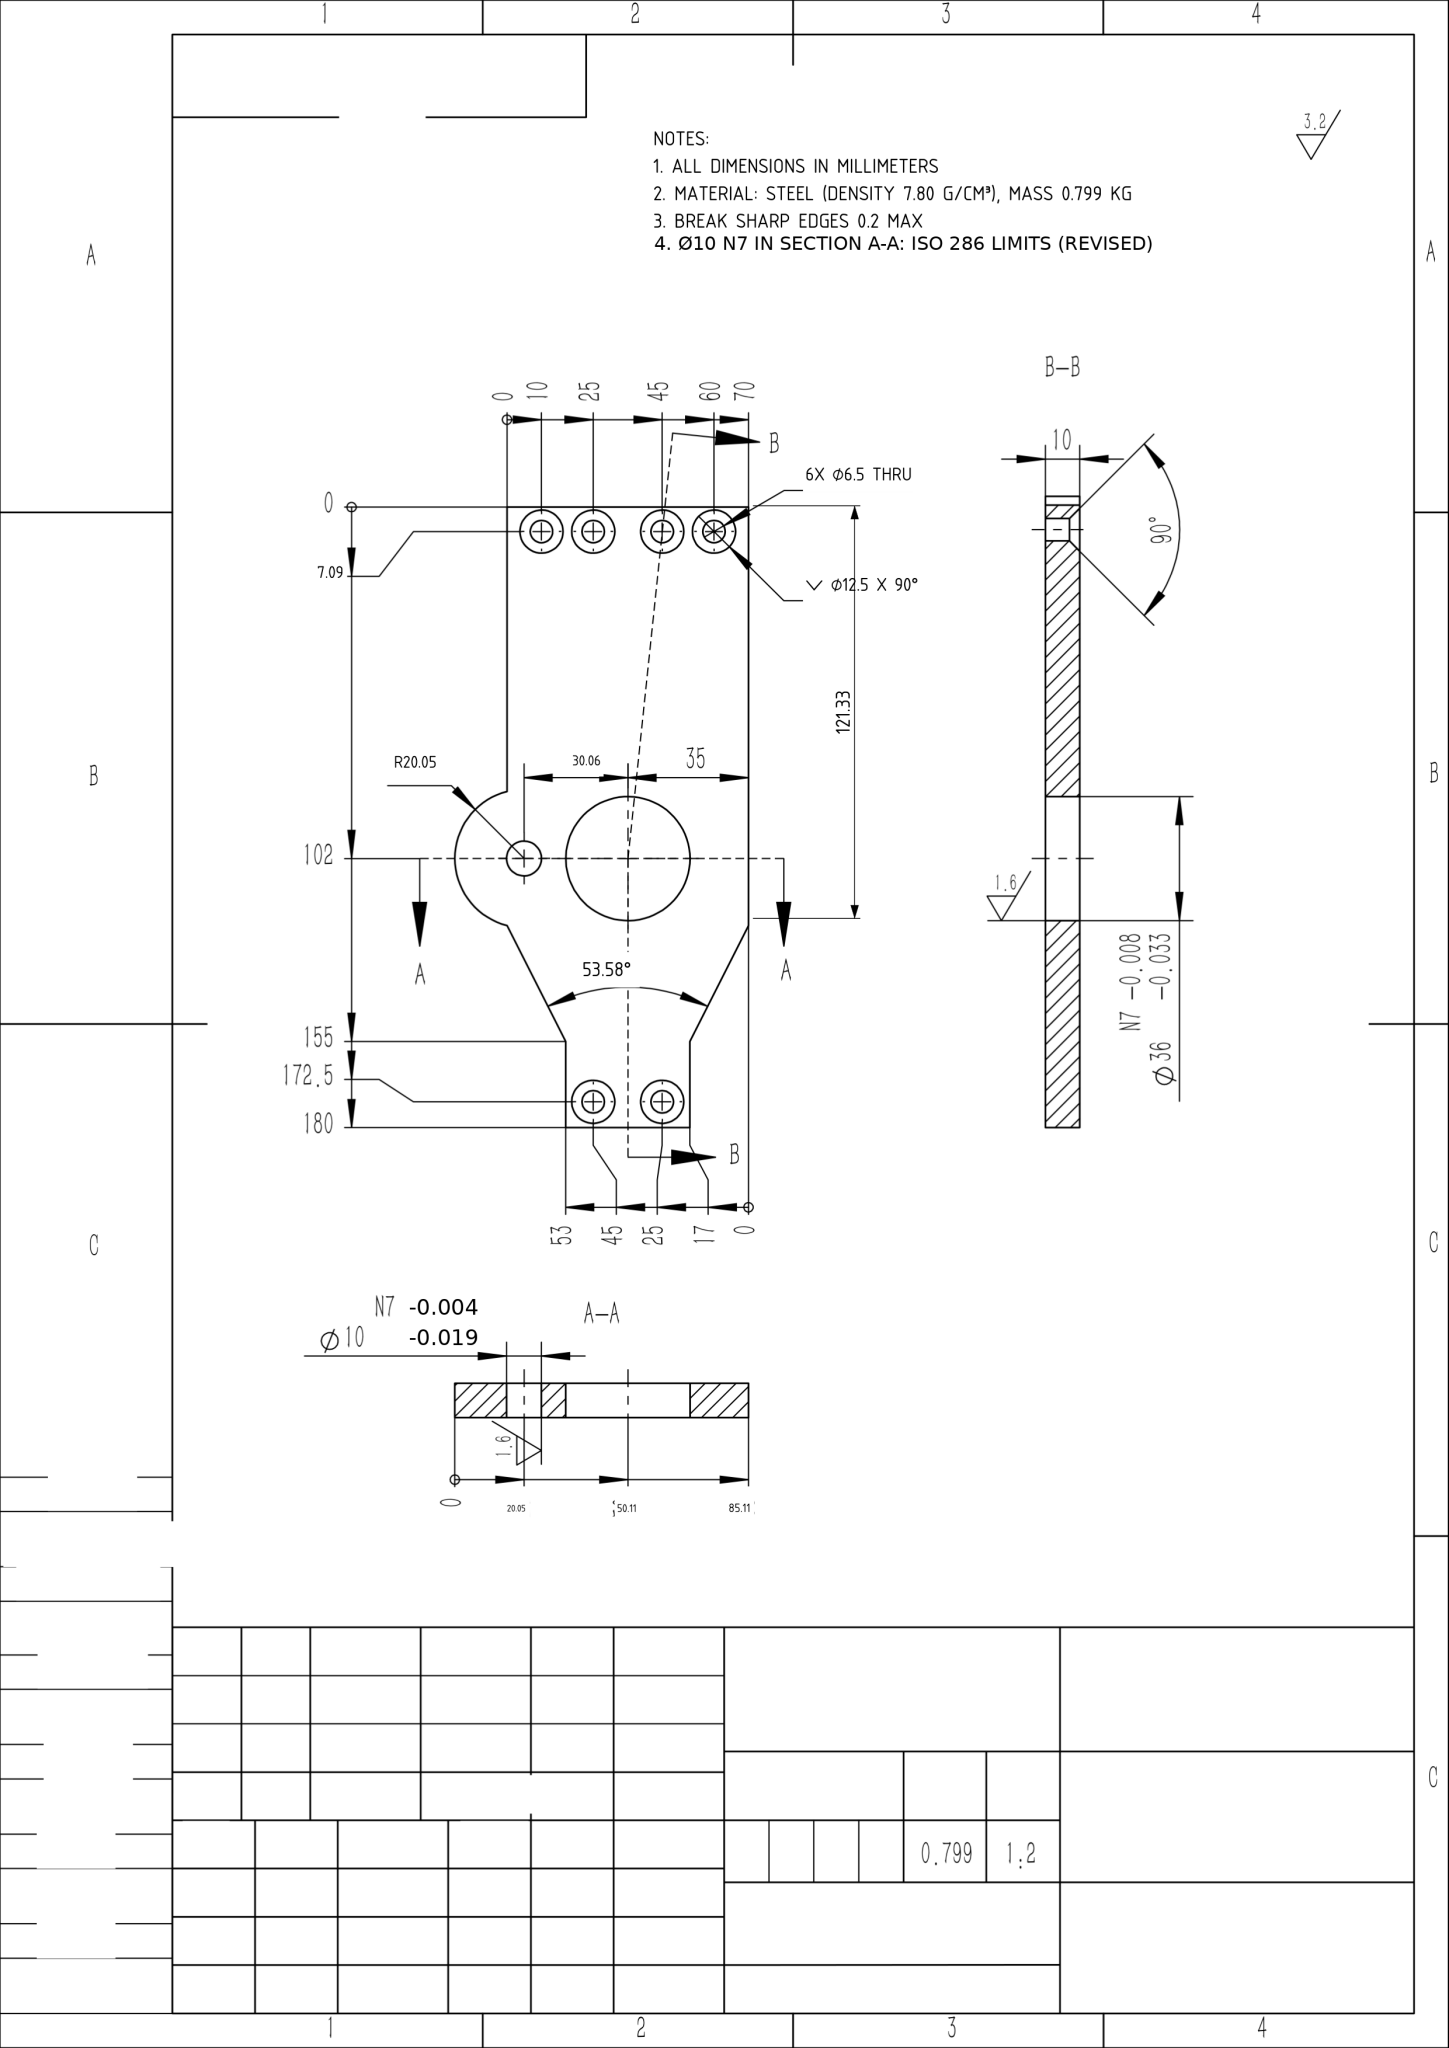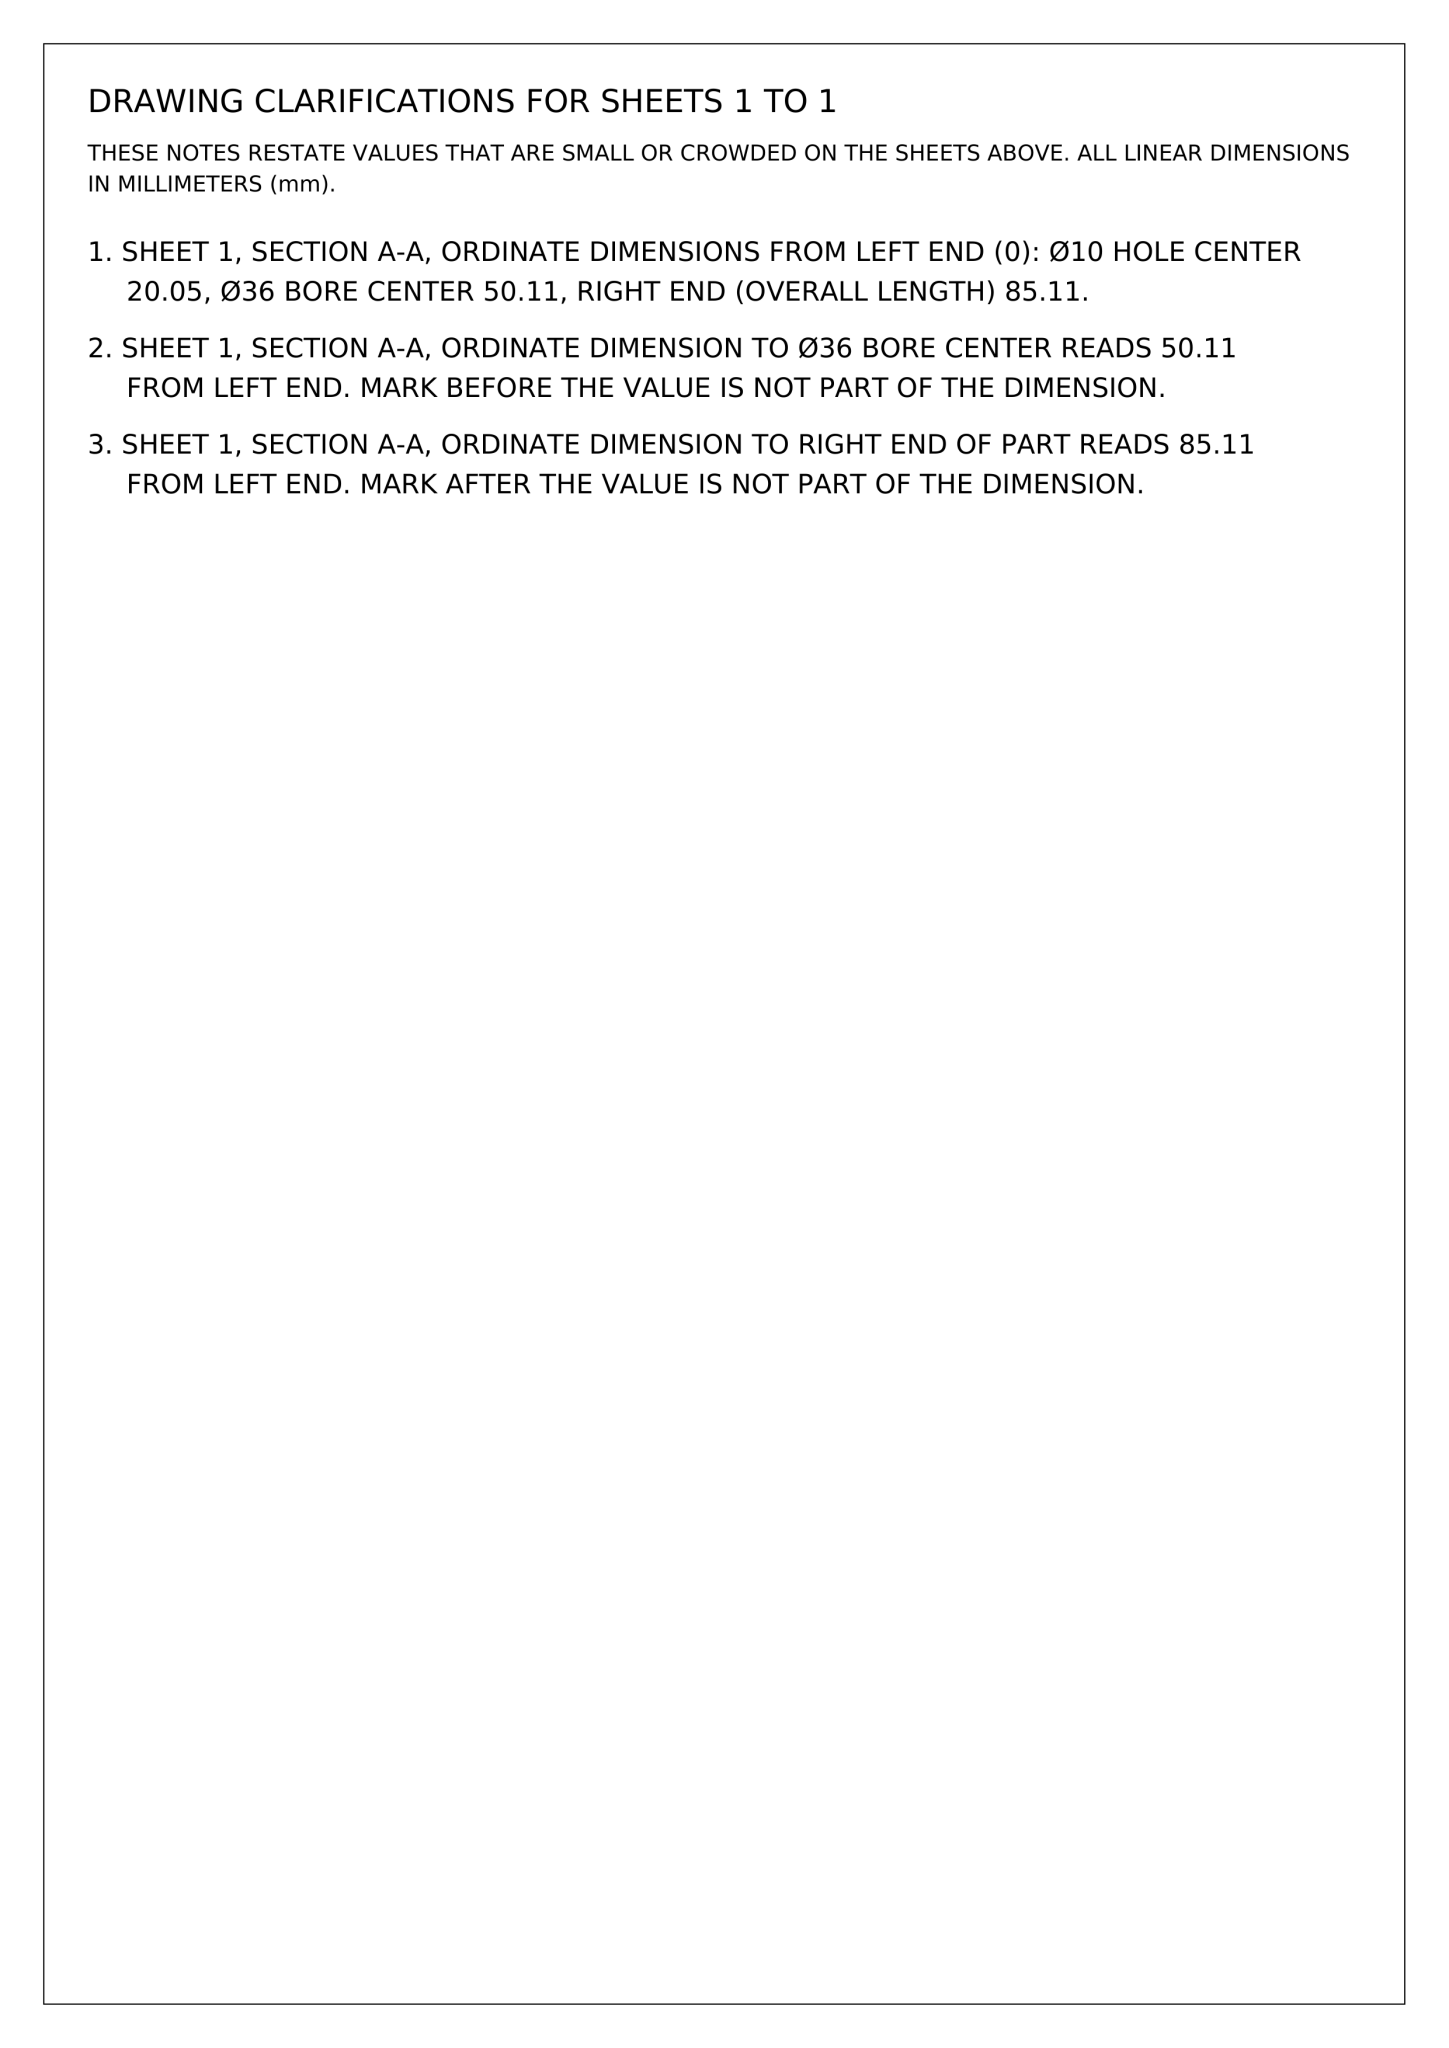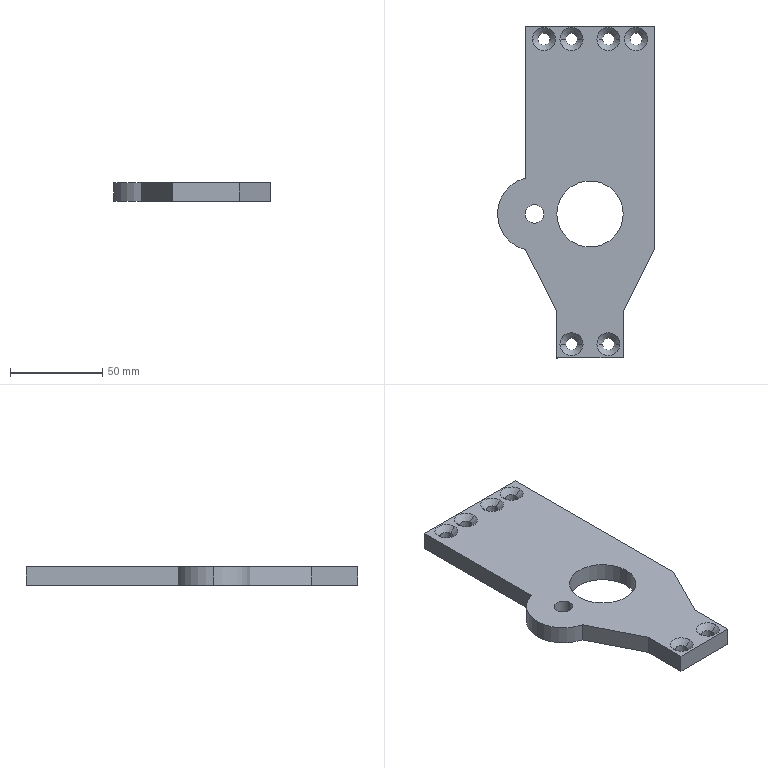Part | NX | mm | 1 solid | 40 faces | box 85.11 x 180 x 10 mm | volume 102438 mm3 | cylinder 18 | cone 12 | plane 10 | commonest cylinder face diameters 6.5 x12 36 x2 10.117 x2 40.117 x2